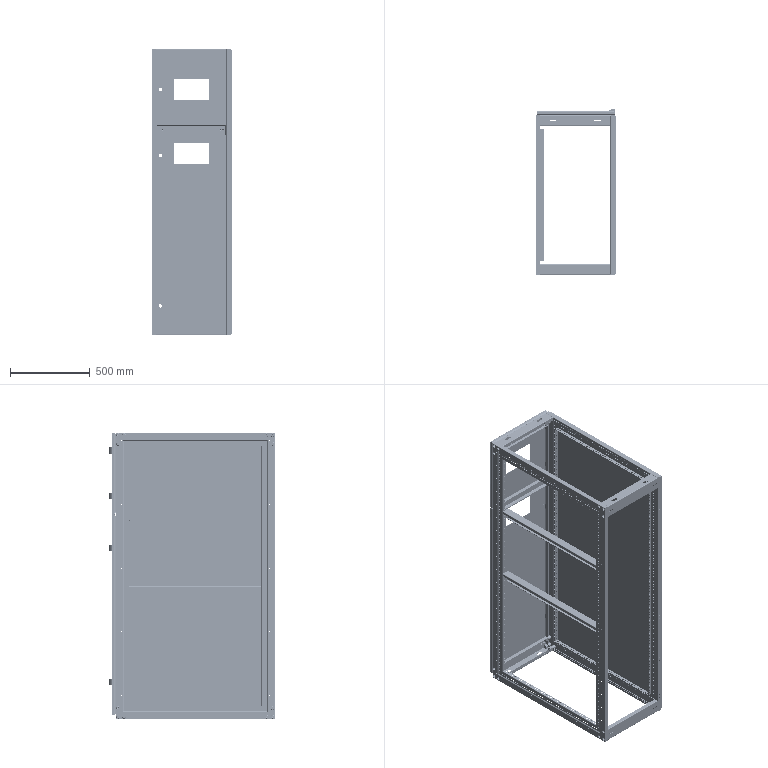Assembly | SolidWorks | mm | 80 component files | 80 solids | 5688 faces | box 508 x 1041.47 x 1800 mm | volume 8275568 mm3 | cylinder 4012 | plane 1276 | spline 216 | cone 184 | commonest cylinder face diameters 9.2 x3028 13.2 x108 22 x104 16 x74 10 x74 7.2 x64 1.473 x58 12 x56
Bill of materials:
500CabinetWidthCrossbeam | 4 | Plain Carbon Steel | Long, thin-walled formed channel. Its open C-type cross-section has unequal legs: a wide top face, one short downturned lip, one tall side wall and a short bottom return flange. The top face has two elongated slots and each end has a group of small round holes.
CrossbeamFixingSleeve | 24 | Plain Carbon Steel | Solid prism with an octagonal end face (a square with chamfered corners) and one round through-bore along the prism axis.
500CabinetWidthDoorCrossbeam | 1 | Plain Carbon Steel | Long, thin-walled C-channel with two equal flanges and radiused bends. Each end of the web has a row of three small round holes.
Connector | 2 |  | Small bent sheet-metal bracket with a stepped (joggled) profile and several bends. A wider flange with four round holes in a line connects through an angled tapered section to a narrower flange with one round hole.
500CabinetWidthLowerDoor | 1 | Plain Carbon Steel | Tall, thin rectangular sheet panel with a rectangular cutout near the top. It has two round holes near one long edge and pairs of small holes near the opposite edge, where the edge also shows small steps or notches.
500CabinetWidthUpperDoor | 1 | Plain Carbon Steel | Roughly square, thin sheet panel with a large central rectangular cutout. It has one polygonal hole near the left edge and two pairs of small round holes near the right edge, which shows segmented steps.
FrameFixingSleeve | 24 |  | Stepped cylindrical sleeve: a larger-diameter body and a smaller-diameter shoulder on the same axis, with a central through-bore and chamfered outer edges.
HighVoltageCabinetHorizontalFrame | 4 | Plain Carbon Steel | Long, straight rail made from a thin-walled formed profile with a constant open cross-section. The section has several bends: a top flange, a vertical web with an inclined offset (jog), a lower vertical segment, a bottom return flange, and a short upturned lip. One face has a dense row of evenly spaced small round holes and another face has a sparser row of small holes. There are larger round holes near both ends, and the ends are cut at angles in steps.
HighVoltageCabinetVerticalFrame | 4 | Plain Carbon Steel | Very long, narrow formed sheet profile with several bends. The cross-section is an open C/hat shape with an inclined jog in one wall and a short return leg. Many rows of small holes run along its length, with larger holes near the ends.
HighVoltageOutletCabinetMountingPlate | 2 | Plain Carbon Steel | Long, thin-walled formed channel with an open C-type profile: a top web, one tall side wall, one short leg and a short bottom return. The tall side wall has one long row of evenly spaced obround slots.
HighVoltageOutletCabinetMountingPlateSideBaffles | 4 | Plain Carbon Steel | Flat rectangular plate with rounded corners and three equal round through-holes in a straight line near one edge.
HighVoltageOuterSealingPlate | 1 | Plain Carbon Steel | Large, thin flat rectangular panel with small holes along both long edges: five evenly spaced holes per side, ten in total.
Hinge1 | 4 |  | Small bent sheet-metal bracket. An L-shaped profile has two round holes in one leg, and the other leg ends in a rolled curl. Its corners are rounded and the curled leg has radiused side cutouts that make it narrower.
Hinge2 | 4 |  | U-shaped bracket made of two parallel flat side plates joined by a rectangular back web. Each side plate has a curved, segment-like outline with a small through-hole near one end and a short tab that turns down at that end with a rounded tip. Two parallel solid cylindrical pins or bosses stick out from the inside of the web, between the side plates.
Mates:
1. coincident | HighVoltageCabinetFrameAssembly-1/HighVoltageCabinetVerticalFrame-2 face at (-1285.437, 151.417, 900.27) dir (-1, 0, 0) | 500CabinetWidthCrossbeamAssembly-1/500CabinetWidthCrossbeam-1 face at (-1285.437, 113.417, 2695.534) dir (1, 0, 0)
2. concentric | HighVoltageCabinetFrameAssembly-1/FrameFixingSleeve-5 edge at (-1294.437, 161.417, 2685.27) dir (1, 0, 0) r 7.5 | 500CabinetWidthCrossbeamAssembly-1/CrossbeamFixingSleeve-2 edge at (-1285.437, 161.417, 2685.27) dir (1, 0, 0) r 8.75
3. parallel | HighVoltageCabinetFrameAssembly-1/HighVoltageCabinetVerticalFrame-2 face at (-1285.437, 176.417, 900.27) dir (0, 1, 0) | 500CabinetWidthCrossbeamAssembly-1/500CabinetWidthCrossbeam-1 face at (-1285.437, 174.417, 2698.27) dir (0, 1, 0)
4. coincident | HighVoltageCabinetFrameAssembly-1/HighVoltageCabinetVerticalFrame-1 face at (-1285.437, -798.583, 2700.27) dir (-1, 0, 0) | 500CabinetWidthCrossbeamAssembly-2/CrossbeamFixingSleeve-4 face at (-1285.437, -782.583, 2674.27) dir (1, 0, 0)
5. concentric | HighVoltageCabinetFrameAssembly-1/FrameFixingSleeve-11 edge at (-1295.437, -808.583, 2685.27) dir (1, 0, 0) r 6 | 500CabinetWidthCrossbeamAssembly-2/CrossbeamFixingSleeve-5 edge at (-1304.937, -808.583, 2685.27) dir (-1, 0, 0) r 4.6
6. parallel | HighVoltageCabinetFrameAssembly-1/HighVoltageCabinetVerticalFrame-1 face at (-1285.437, -823.583, 2700.27) dir (0, -1, 0) | 500CabinetWidthCrossbeamAssembly-2/500CabinetWidthCrossbeam-1 face at (-1725.437, -821.583, 2698.27) dir (0, -1, 0)
7. concentric | HighVoltageCabinetFrameAssembly-1/FrameFixingSleeve-1 edge at (-1294.437, 161.417, 915.27) dir (1, 0, 0) r 7.5 | 500CabinetWidthCrossbeamAssembly-3/CrossbeamFixingSleeve-5 edge at (-1285.437, 161.417, 915.27) dir (1, 0, 0) r 8.75
8. coincident | HighVoltageCabinetFrameAssembly-1/HighVoltageCabinetHorizontalFrame-1 face at (-1285.437, -823.583, 925.27) dir (-1, 0, 0) | 500CabinetWidthCrossbeamAssembly-3/CrossbeamFixingSleeve-5 face at (-1285.437, 172.417, 926.27) dir (1, 0, 0)
9. parallel | HighVoltageCabinetFrameAssembly-1/HighVoltageCabinetHorizontalFrame-1 face at (-1285.437, -823.583, 900.27) dir (0, 0, -1) | 500CabinetWidthCrossbeamAssembly-3/500CabinetWidthCrossbeam-1 face at (-1725.437, 174.417, 902.27) dir (0, 0, -1)
10. coincident | HighVoltageCabinetFrameAssembly-1/HighVoltageCabinetVerticalFrame-1 face at (-1285.437, -798.583, 2700.27) dir (-1, 0, 0) | 500CabinetWidthCrossbeamAssembly-4/CrossbeamFixingSleeve-2 face at (-1285.437, -819.583, 904.27) dir (1, 0, 0)
11. concentric | HighVoltageCabinetFrameAssembly-1/FrameFixingSleeve-8 edge at (-1295.437, -808.583, 915.27) dir (1, 0, 0) r 6 | 500CabinetWidthCrossbeamAssembly-4/CrossbeamFixingSleeve-2 edge at (-1304.937, -808.583, 915.27) dir (-1, 0, 0) r 4.6
12. parallel | HighVoltageCabinetFrameAssembly-1/HighVoltageCabinetHorizontalFrame-1 face at (-1285.437, -823.583, 900.27) dir (0, 0, -1) | 500CabinetWidthCrossbeamAssembly-4/500CabinetWidthCrossbeam-1 face at (-1285.437, -821.583, 902.27) dir (0, 0, -1)
13. coincident | 500CabinetWidthCrossbeamAssembly-3/CrossbeamFixingSleeve-1 face at (-1725.437, 172.417, 959.27) dir (-1, 0, 0) | HighVoltageCabinetFrameAssembly-2/HighVoltageCabinetVerticalFrame-2 face at (-1725.437, 151.417, 2700.27) dir (1, 0, 0)
14. concentric | 500CabinetWidthCrossbeamAssembly-3/CrossbeamFixingSleeve-2 face at (-1714.437, 161.417, 915.27) dir (-1, 0, 0) r 8.75 | HighVoltageCabinetFrameAssembly-2/FrameFixingSleeve-5 face at (-1755.437, 161.417, 915.27) dir (-1, 0, 0) r 9
15. parallel | 500CabinetWidthCrossbeamAssembly-3/500CabinetWidthCrossbeam-1 face at (-1725.437, 174.417, 902.27) dir (0, 1, 0) | HighVoltageCabinetFrameAssembly-2/HighVoltageCabinetVerticalFrame-2 face at (-1725.437, 176.417, 2700.27) dir (0, 1, 0)
16. coincident | HighVoltageCabinetFrameAssembly-1/HighVoltageCabinetVerticalFrame-2 face at (-1285.437, 176.417, 900.27) dir (0, 1, 0) | 500CabinetWidthDoorCrossbeamAssembly-1/500CabinetWidthDoorCrossbeam-1 face at (-1285.437, 176.417, 2220.27) dir (0, 1, 0)
17. distance | 500CabinetWidthDoorCrossbeamAssembly-1/500CabinetWidthDoorCrossbeam-1 face at (-1285.437, 151.417, 2220.27) dir (0, 0, 1) | HighVoltageCabinetFrameAssembly-1/HighVoltageCabinetHorizontalFrame-2 face at (-1285.437, 176.417, 2700.27) dir (0, 0, 1)
18. coincident | HighVoltageCabinetFrameAssembly-2/HighVoltageCabinetVerticalFrame-2 face at (-1725.437, 151.417, 2700.27) dir (1, 0, 0) | 500CabinetWidthDoorCrossbeamAssembly-1/500CabinetWidthDoorCrossbeam-1 face at (-1725.437, 174.417, 2217.534) dir (-1, 0, 0)
19. coincident | HighVoltageCabinetFrameAssembly-1/HighVoltageCabinetVerticalFrame-2 face at (-1285.437, 176.417, 900.27) dir (0, 1, 0) | Hinge1-1 face at (-1281.937, 176.417, 2608.02) dir (0, -1, 0)
20. concentric | HighVoltageCabinetFrameAssembly-1/HighVoltageCabinetVerticalFrame-2 edge at (-1272.937, 176.417, 2600.77) dir (0, 1, 0) r 3.6 | Hinge1-1 edge at (-1272.937, 179.417, 2600.77) dir (0, 1, 0) r 3.75
21. coincident | HighVoltageCabinetFrameAssembly-1/HighVoltageCabinetVerticalFrame-2 face at (-1255.437, 176.417, 900.27) dir (1, 0, 0) | Hinge1-1 face at (-1255.437, 182.417, 2608.02) dir (1, 0, 0)
22. coincident | HighVoltageCabinetFrameAssembly-1/HighVoltageCabinetVerticalFrame-2 face at (-1285.437, 176.417, 900.27) dir (0, 1, 0) | Hinge1-2 face at (-1281.937, 176.417, 2321.52) dir (0, -1, 0)
23. concentric | HighVoltageCabinetFrameAssembly-1/HighVoltageCabinetVerticalFrame-2 edge at (-1272.937, 176.417, 2314.27) dir (0, 1, 0) r 3.6 | Hinge1-2 edge at (-1272.937, 179.417, 2314.27) dir (0, 1, 0) r 3.75
24. coincident | HighVoltageCabinetFrameAssembly-1/HighVoltageCabinetVerticalFrame-2 face at (-1255.437, 176.417, 900.27) dir (1, 0, 0) | Hinge1-2 face at (-1255.437, 182.417, 2321.52) dir (1, 0, 0)
25. coincident | HighVoltageCabinetFrameAssembly-1/HighVoltageCabinetVerticalFrame-2 face at (-1285.437, 176.417, 900.27) dir (0, 1, 0) | Hinge1-3 face at (-1281.937, 176.417, 1996.52) dir (0, -1, 0)
26. concentric | HighVoltageCabinetFrameAssembly-1/HighVoltageCabinetVerticalFrame-2 edge at (-1272.937, 176.417, 1989.27) dir (0, 1, 0) r 3.6 | Hinge1-3 edge at (-1272.937, 179.417, 1989.27) dir (0, 1, 0) r 3.75
27. coincident | HighVoltageCabinetFrameAssembly-1/HighVoltageCabinetVerticalFrame-2 face at (-1255.437, 176.417, 900.27) dir (1, 0, 0) | Hinge1-3 face at (-1255.437, 182.417, 1996.52) dir (1, 0, 0)
28. coincident | HighVoltageCabinetFrameAssembly-1/HighVoltageCabinetVerticalFrame-2 face at (-1285.437, 176.417, 900.27) dir (0, 1, 0) | Hinge1-4 face at (-1281.937, 176.417, 1156.02) dir (0, -1, 0)
29. concentric | HighVoltageCabinetFrameAssembly-1/HighVoltageCabinetVerticalFrame-2 edge at (-1272.937, 176.417, 1148.77) dir (0, 1, 0) r 3.6 | Hinge1-4 edge at (-1272.937, 179.417, 1148.77) dir (0, 1, 0) r 3.75
30. coincident | HighVoltageCabinetFrameAssembly-1/HighVoltageCabinetVerticalFrame-2 face at (-1255.437, 176.417, 900.27) dir (1, 0, 0) | Hinge1-4 face at (-1255.437, 182.417, 1156.02) dir (1, 0, 0)
31. coincident | Hinge1-1 face at (-1261.437, 182.417, 2608.02) dir (0, 0, 1) | Hinge2-1 face at (-1270.557, 188.93, 2608.02) dir (0, 0, 1)
32. concentric | Hinge1-1 edge at (-1260.937, 210.917, 2603.02) dir (0, 0, 1) r 2.5 | Hinge2-1 edge at (-1260.937, 210.917, 2608.02) dir (0, 0, 1) r 2.75
33. coincident | Hinge1-2 face at (-1261.437, 182.417, 2321.52) dir (0, 0, 1) | Hinge2-2 face at (-1270.557, 188.93, 2321.52) dir (0, 0, 1)
34. concentric | Hinge1-2 edge at (-1260.937, 210.917, 2316.52) dir (0, 0, 1) r 2.5 | Hinge2-2 edge at (-1260.937, 210.917, 2321.52) dir (0, 0, 1) r 2.75
35. coincident | Hinge1-3 face at (-1261.437, 182.417, 1996.52) dir (0, 0, 1) | Hinge2-3 face at (-1270.571, 188.936, 1996.52) dir (0, 0, 1)
36. concentric | Hinge1-3 edge at (-1260.937, 210.917, 1991.52) dir (0, 0, 1) r 2.5 | Hinge2-3 edge at (-1260.937, 210.917, 1996.52) dir (0, 0, 1) r 2.75
37. coincident | Hinge1-4 face at (-1261.437, 182.417, 1156.02) dir (0, 0, 1) | Hinge2-4 face at (-1270.571, 188.936, 1156.02) dir (0, 0, 1)
38. concentric | Hinge1-4 edge at (-1260.937, 210.917, 1151.02) dir (0, 0, 1) r 2.5 | Hinge2-4 edge at (-1260.937, 210.917, 1156.02) dir (0, 0, 1) r 2.75
39. coincident | Hinge2-3 face at (-1296.441, 201.932, 1996.52) dir (-0.0004256, -1, 0) | Hinge2-4 face at (-1296.441, 201.932, 1156.02) dir (-0.0004256, -1, 0)
40. coincident | Hinge2-1 face at (-1296.435, 201.91, 2608.02) dir (0.0002055, -1, 0) | Hinge2-2 face at (-1296.435, 201.91, 2321.52) dir (0.0002055, -1, 0)
41. coincident | Hinge2-1 face at (-1296.435, 201.91, 2608.02) dir (0.0002055, -1, 0) | 500CabinetWidthUpperDoor-1 face at (-1259.435, 201.917, 2191.77) dir (-0.0002055, 1, 0)
42. concentric | 500CabinetWidthUpperDoor-1 edge at (-1281.435, 200.413, 2594.27) dir (-0.0002055, 1, 0) r 4.75 | Hinge2-1 edge at (-1281.435, 200.913, 2594.27) dir (0.0002055, -1, 0) r 4.75
43. parallel | 500CabinetWidthCrossbeamAssembly-1/500CabinetWidthCrossbeam-1 face at (-1285.437, 174.417, 2698.27) dir (0, 0, 1) | 500CabinetWidthUpperDoor-1 face at (-1259.435, 201.917, 2698.27) dir (0, 0, 1)
44. coincident | Hinge2-3 face at (-1296.441, 201.932, 1996.52) dir (-0.0004256, -1, 0) | 500CabinetWidthLowerDoor-1 face at (-1259.441, 201.916, 924.27) dir (0.0004256, 1, 0)
45. concentric | Hinge2-3 edge at (-1281.441, 200.926, 1982.77) dir (-0.0004256, -1, 0) r 4.75 | 500CabinetWidthLowerDoor-1 edge at (-1281.441, 200.426, 1982.77) dir (0.0004256, 1, 0) r 4.75
46. parallel | HighVoltageCabinetFrameAssembly-1/HighVoltageCabinetHorizontalFrame-2 face at (-1285.437, 176.417, 2700.27) dir (0, 0, 1) | 500CabinetWidthLowerDoor-1 face at (-1259.441, 201.916, 2188.77) dir (0, 0, 1)
47. coincident | HighVoltageMountingPlateAssembly-1/HighVoltageOutletCabinetMountingPlateSideBaffles-1 face at (-1702.937, 91.417, 2147.77) dir (0, 1, 0) | HighVoltageCabinetFrameAssembly-2/HighVoltageCabinetVerticalFrame-2 face at (-1750.437, 91.417, 2700.27) dir (0, -1, 0)
48. concentric | HighVoltageCabinetFrameAssembly-2/HighVoltageCabinetVerticalFrame-2 edge at (-1735.437, 91.417, 2200.27) dir (0, -1, 0) r 4.6 | HighVoltageMountingPlateAssembly-1/HighVoltageOutletCabinetMountingPlateSideBaffles-1 edge at (-1735.437, 91.417, 2200.27) dir (0, 1, 0) r 4.75
49. parallel | 500CabinetWidthDoorCrossbeamAssembly-1/500CabinetWidthDoorCrossbeam-1 face at (-1285.437, 151.417, 2220.27) dir (0, 0, 1) | HighVoltageMountingPlateAssembly-1/HighVoltageOutletCabinetMountingPlate-1 face at (-1700.437, 91.417, 2215.27) dir (0, 0, 1)
50. coincident | HighVoltageCabinetFrameAssembly-2/HighVoltageCabinetVerticalFrame-2 face at (-1750.437, 91.417, 2700.27) dir (0, -1, 0) | HighVoltageMountingPlateAssembly-2/HighVoltageOutletCabinetMountingPlateSideBaffles-1 face at (-1702.937, 91.417, 1667.77) dir (0, 1, 0)
51. concentric | HighVoltageCabinetFrameAssembly-2/HighVoltageCabinetVerticalFrame-2 edge at (-1735.437, 91.417, 1720.27) dir (0, -1, 0) r 4.6 | HighVoltageMountingPlateAssembly-2/HighVoltageOutletCabinetMountingPlateSideBaffles-1 edge at (-1735.437, 91.417, 1720.27) dir (0, 1, 0) r 4.75
52. parallel | HighVoltageMountingPlateAssembly-1/HighVoltageOutletCabinetMountingPlate-1 face at (-1700.437, 91.417, 2215.27) dir (0, 0, 1) | HighVoltageMountingPlateAssembly-2/HighVoltageOutletCabinetMountingPlate-1 face at (-1700.437, 91.417, 1735.27) dir (0, 0, 1)
53. coincident | HighVoltageCabinetFrameAssembly-1/HighVoltageCabinetHorizontalFrame-2 face at (-1255.437, 176.417, 2700.27) dir (1, 0, 0) | HighVoltageOuterSealingPlate-1 face at (-1255.437, 9121.417, 2695.27) dir (-1, 0, 0)
54. concentric | HighVoltageCabinetFrameAssembly-1/HighVoltageCabinetVerticalFrame-1 edge at (-1255.437, -788.583, 2650.27) dir (1, 0, 0) r 4.6 | HighVoltageOuterSealingPlate-1 edge at (-1252.437, -788.583, 2650.27) dir (-1, 0, 0) r 3.5
55. parallel | HighVoltageCabinetFrameAssembly-1/HighVoltageCabinetHorizontalFrame-2 face at (-1285.437, 176.417, 2700.27) dir (0, 0, 1) | HighVoltageOuterSealingPlate-1 face at (-1255.437, 9121.417, 2695.27) dir (0, 0, 1)
56. coincident | 500CabinetWidthCrossbeam-1 face at (-33.665, 33.973, 660) dir (0, 0, 1) | CrossbeamFixingSleeve-1 face at (-33.665, 12.709, 660) dir (0, 0, 1)
57. coincident | 500CabinetWidthCrossbeam-1 face at (-33.665, -44.291, 660) dir (1, 0, 0) | CrossbeamFixingSleeve-1 face at (-33.665, 16.209, 660) dir (-1, 0, 0)
58. coincident | 500CabinetWidthCrossbeam-1 face at (-35.665, 34.709, 660) dir (0, -1, 0) | CrossbeamFixingSleeve-1 face at (-30.165, 34.709, 660) dir (0, 1, 0)
59. coincident | 500CabinetWidthCrossbeam-1 face at (-32.928, -42.291, 660) dir (0, 0, 1) | CrossbeamFixingSleeve-2 face at (-33.665, -42.291, 660) dir (0, 0, 1)
60. coincident | 500CabinetWidthCrossbeam-1 face at (-33.665, -44.291, 660) dir (1, 0, 0) | CrossbeamFixingSleeve-2 face at (-33.665, -38.791, 660) dir (-1, 0, 0)
61. coincident | 500CabinetWidthCrossbeam-1 face at (-35.665, -42.291, 660) dir (0, 1, 0) | CrossbeamFixingSleeve-2 face at (-30.165, -42.291, 660) dir (0, -1, 0)
62. coincident | 500CabinetWidthCrossbeam-1 face at (-35.665, -42.291, 660) dir (0, 1, 0) | CrossbeamFixingSleeve-3 face at (6.835, -42.291, 660) dir (0, -1, 0)
63. coincident | 500CabinetWidthCrossbeam-1 face at (-32.928, 33.973, 660) dir (0, 0, 1) | CrossbeamFixingSleeve-3 face at (3.335, -42.291, 660) dir (0, 0, 1)
64. coincident | 500CabinetWidthCrossbeam-1 face at (25.335, -44.291, 660) dir (-1, 0, 0) | CrossbeamFixingSleeve-3 face at (25.335, -38.791, 660) dir (1, 0, 0)
65. coincident | 500CabinetWidthDoorCrossbeam-1 face at (-118.393, 199.408, 470) dir (1, 0, 0) | Connector-1 face at (-118.393, 191.908, 400) dir (-1, 0, 0)
66. concentric | 500CabinetWidthDoorCrossbeam-1 edge at (-118.393, 178.408, 440) dir (-1, 0, 0) r 4.6 | Connector-1 edge at (-116.393, 178.408, 440) dir (-1, 0, 0) r 4.5
67. parallel | 500CabinetWidthDoorCrossbeam-1 face at (-120.393, 199.408, 410) dir (0, 0, -1) | Connector-1 face at (-90.393, 246.908, 415) dir (0, 0, -1)
68. coincident | 500CabinetWidthDoorCrossbeam-1 face at (-118.393, 199.408, 470) dir (1, 0, 0) | Connector-2 face at (-118.393, -233.092, 480) dir (-1, 0, 0)
69. concentric | 500CabinetWidthDoorCrossbeam-1 edge at (-118.393, -219.592, 440) dir (-1, 0, 0) r 4.6 | Connector-2 edge at (-116.393, -219.592, 440) dir (-1, 0, 0) r 4.5
70. parallel | 500CabinetWidthDoorCrossbeam-1 face at (-120.393, 199.408, 410) dir (0, 0, -1) | Connector-2 face at (-115.393, -233.092, 400) dir (0, 0, -1)
71. coincident | HighVoltageCabinetVerticalFrame-1 face at (-27.582, -40.091, 896) dir (0, 0.7071, -0.7071) | HighVoltageCabinetHorizontalFrame-1 face at (-29.582, -40.091, 896) dir (0, -0.7071, 0.7071)
72. coincident | HighVoltageCabinetVerticalFrame-1 face at (-27.582, -40.091, 2696) dir (1, 0, 0) | HighVoltageCabinetHorizontalFrame-1 face at (-27.582, -40.091, 896) dir (1, 0, 0)
73. coincident | HighVoltageCabinetVerticalFrame-1 edge at (-27.582, -25.091, 911) dir (1, 0, 0) r 11 | HighVoltageCabinetHorizontalFrame-1 edge at (-27.582, -25.091, 911) dir (1, 0, 0) r 11
74. coincident | HighVoltageCabinetHorizontalFrame-1 face at (-27.582, -40.091, 896) dir (1, 0, 0) | HighVoltageCabinetVerticalFrame-2 face at (-27.582, 959.909, 896) dir (1, 0, 0)
75. coincident | HighVoltageCabinetHorizontalFrame-1 face at (-27.582, 459.909, 1396) dir (0, 0.7071, 0.7071) | HighVoltageCabinetVerticalFrame-2 face at (-29.582, 959.909, 896) dir (0, -0.7071, -0.7071)
76. coincident | HighVoltageCabinetHorizontalFrame-1 edge at (-27.582, 944.909, 911) dir (1, 0, 0) r 11 | HighVoltageCabinetVerticalFrame-2 edge at (-27.582, 944.909, 911) dir (-1, 0, 0) r 11
77. coincident | HighVoltageCabinetVerticalFrame-2 face at (-27.582, 959.909, 896) dir (1, 0, 0) | HighVoltageCabinetHorizontalFrame-2 face at (-27.582, 959.909, 2696) dir (1, 0, 0)
78. coincident | HighVoltageCabinetVerticalFrame-2 face at (-27.582, 959.909, 2696) dir (0, -0.7071, 0.7071) | HighVoltageCabinetHorizontalFrame-2 face at (-29.582, 959.909, 2696) dir (0, 0.7071, -0.7071)
79. coincident | HighVoltageCabinetVerticalFrame-2 edge at (-27.582, 944.909, 2681) dir (1, 0, 0) r 11 | HighVoltageCabinetHorizontalFrame-2 edge at (-27.582, 944.909, 2681) dir (1, 0, 0) r 11
80. coincident | HighVoltageCabinetHorizontalFrame-1 face at (-27.582, -40.091, 896) dir (1, 0, 0) | FrameFixingSleeve-1 face at (-27.582, 935.911, 910.826) dir (1, 0, 0)
81. concentric | HighVoltageCabinetHorizontalFrame-1 edge at (-27.582, 944.909, 911) dir (1, 0, 0) r 11 | FrameFixingSleeve-1 edge at (-27.582, 944.909, 911) dir (1, 0, 0) r 9
82. coincident | HighVoltageCabinetHorizontalFrame-1 face at (-27.582, -40.091, 896) dir (1, 0, 0) | FrameFixingSleeve-2 face at (-27.582, 900.247, 915.721) dir (1, 0, 0)
83. concentric | HighVoltageCabinetHorizontalFrame-1 edge at (-27.582, 907.909, 911) dir (1, 0, 0) r 11 | FrameFixingSleeve-2 edge at (-27.582, 907.909, 911) dir (1, 0, 0) r 9
84. coincident | HighVoltageCabinetVerticalFrame-2 face at (-27.582, 959.909, 896) dir (1, 0, 0) | FrameFixingSleeve-3 face at (-27.582, 936.074, 967.712) dir (1, 0, 0)
85. concentric | HighVoltageCabinetVerticalFrame-2 edge at (-27.582, 944.909, 966) dir (-1, 0, 0) r 11 | FrameFixingSleeve-3 edge at (-27.582, 944.909, 966) dir (1, 0, 0) r 10
86. coincident | HighVoltageOutletCabinetMountingPlate-1 face at (-73.445, 38.473, 1260) dir (0, 0, 1) | HighVoltageOutletCabinetMountingPlateSideBaffles-1 face at (-72.945, -26.027, 1260) dir (0, 0, 1)
87. distance | HighVoltageOutletCabinetMountingPlateSideBaffles-1 face at (-72.945, 38.973, 1258) dir (0, 1, 0) | HighVoltageOutletCabinetMountingPlate-1 face at (-75.445, 39.473, 1260) dir (0, -1, 0)
88. distance | HighVoltageOutletCabinetMountingPlateSideBaffles-1 face at (-72.945, -26.027, 1258) dir (-1, 0, 0) | HighVoltageOutletCabinetMountingPlate-1 face at (-73.445, -28.527, 1260) dir (1, 0, 0)
89. coincident | HighVoltageOutletCabinetMountingPlate-1 face at (-28.445, 41.473, 430) dir (0, 0, -1) | HighVoltageOutletCabinetMountingPlateSideBaffles-2 face at (-72.945, -26.027, 430) dir (0, 0, -1)
90. distance | HighVoltageOutletCabinetMountingPlateSideBaffles-2 face at (-72.945, 38.973, 430) dir (0, 1, 0) | HighVoltageOutletCabinetMountingPlate-1 face at (-75.445, 39.473, 1260) dir (0, -1, 0)
91. distance | HighVoltageOutletCabinetMountingPlateSideBaffles-2 face at (-27.945, -26.027, 430) dir (1, 0, 0) | HighVoltageOutletCabinetMountingPlate-1 face at (-27.445, 41.473, 1260) dir (-1, 0, 0)